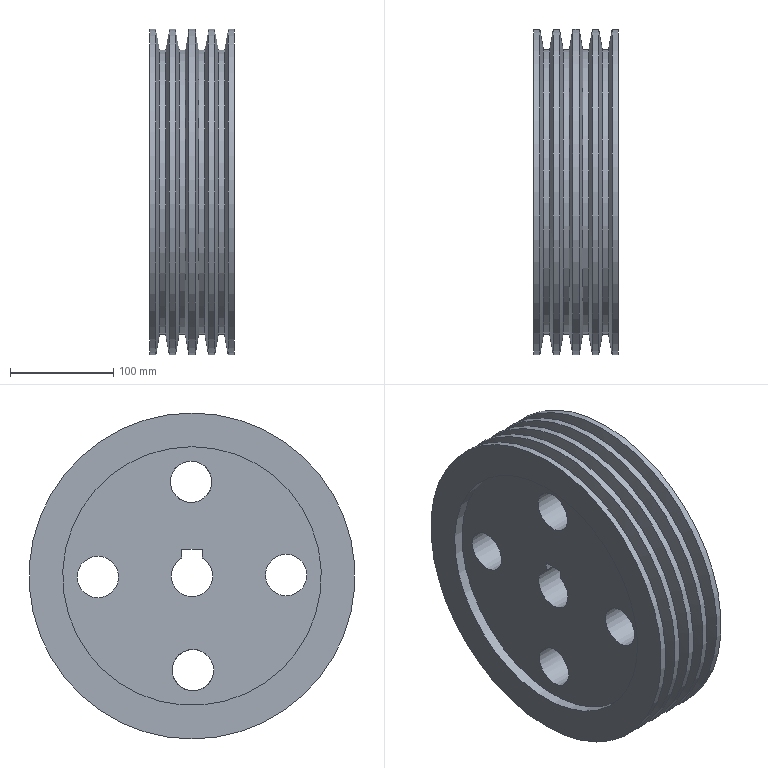Component | NX | LARGE_PULLEY_2 | 1 solid | 31 faces | volume 4297038 mm3 | cylinder 16 | cone 8 | plane 7 | commonest cylinder face diameters 40 x5 315 x5 275.608 x4 250 x2